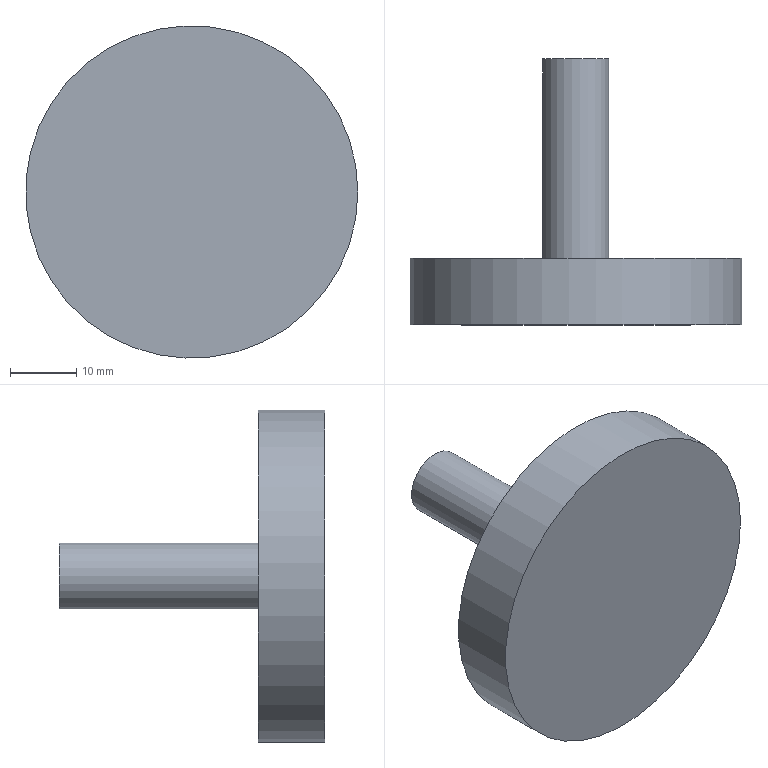Component | NX | BASE_PLATE | 1 solid | 5 faces | box 50 x 40 x 50 mm | volume 21991 mm3 | plane 3 | cylinder 2 | commonest cylinder face diameters 50 x1 10 x1
STEP:
#1=CARTESIAN_POINT('',(0.,0.,0.));
#2=DIRECTION('',(0.,0.,1.));
#3=DIRECTION('',(1.,0.,0.));
#4=AXIS2_PLACEMENT_3D('',#1,#2,#3);
#5=CARTESIAN_POINT('',(25.,-10.,-0.));
#6=VERTEX_POINT('',#5);
#7=CARTESIAN_POINT('',(0.,-10.,0.));
#8=DIRECTION('',(0.,-1.,0.));
#9=DIRECTION('',(1.,0.,-0.));
#10=AXIS2_PLACEMENT_3D('',#7,#8,#9);
#11=CIRCLE('',#10,25.);
#12=CARTESIAN_POINT('',(0.,-10.,0.));
#13=DIRECTION('',(0.,1.,0.));
#14=DIRECTION('',(0.,0.,1.));
#15=AXIS2_PLACEMENT_3D('',#12,#13,#14);
#16=CYLINDRICAL_SURFACE('',#15,25.);
#17=CARTESIAN_POINT('',(7.854,0.));
#18=DIRECTION('',(-1.,0.));
#19=VECTOR('',#18,1.);
#20=LINE('',#17,#19);
#21=(GEOMETRIC_REPRESENTATION_CONTEXT(2)PARAMETRIC_REPRESENTATION_CONTEXT()REPRESENTATION_CONTEXT('',''));
#22=DEFINITIONAL_REPRESENTATION('',(#20),#21);
#23=PCURVE('',#16,#22);
#24=CARTESIAN_POINT('',(0.,-10.,0.));
#25=DIRECTION('',(0.,-1.,0.));
#26=DIRECTION('',(0.,0.,-1.));
#27=AXIS2_PLACEMENT_3D('',#24,#25,#26);
#28=PLANE('',#27);
#29=CARTESIAN_POINT('',(0.,0.));
#30=DIRECTION('',(0.,1.));
#31=AXIS2_PLACEMENT_2D('',#29,#30);
#32=CIRCLE('',#31,25.);
#33=(GEOMETRIC_REPRESENTATION_CONTEXT(2)PARAMETRIC_REPRESENTATION_CONTEXT()REPRESENTATION_CONTEXT('',''));
#34=DEFINITIONAL_REPRESENTATION('',(#32),#33);
#35=PCURVE('',#28,#34);
#36=SURFACE_CURVE('',#11,(#23,#35),.PCURVE_S1.);
#37=EDGE_CURVE('',#6,#6,#36,.T.);
#38=ORIENTED_EDGE('',*,*,#37,.F.);
#39=CARTESIAN_POINT('',(25.,0.,-0.));
#40=VERTEX_POINT('',#39);
#41=CARTESIAN_POINT('',(25.,-10.,0.));
#42=CARTESIAN_POINT('',(25.,0.,0.));
#43=B_SPLINE_CURVE_WITH_KNOTS('',1,(#41,#42),.UNSPECIFIED.,.F.,.F.,(2,2),(0.,10.),.PIECEWISE_BEZIER_KNOTS.);
#44=CARTESIAN_POINT('',(7.854,0.));
#45=DIRECTION('',(0.,1.));
#46=VECTOR('',#45,1.);
#47=LINE('',#44,#46);
#48=(GEOMETRIC_REPRESENTATION_CONTEXT(2)PARAMETRIC_REPRESENTATION_CONTEXT()REPRESENTATION_CONTEXT('',''));
#49=DEFINITIONAL_REPRESENTATION('',(#47),#48);
#50=PCURVE('',#16,#49);
#51=CARTESIAN_POINT('',(1.571,0.));
#52=DIRECTION('',(0.,1.));
#53=VECTOR('',#52,1.);
#54=LINE('',#51,#53);
#55=(GEOMETRIC_REPRESENTATION_CONTEXT(2)PARAMETRIC_REPRESENTATION_CONTEXT()REPRESENTATION_CONTEXT('',''));
#56=DEFINITIONAL_REPRESENTATION('',(#54),#55);
#57=PCURVE('',#16,#56);
#58=SEAM_CURVE('',#43,(#50,#57),.PCURVE_S1.);
#59=EDGE_CURVE('',#6,#40,#58,.T.);
#60=ORIENTED_EDGE('',*,*,#59,.T.);
#61=CARTESIAN_POINT('',(0.,0.,0.));
#62=DIRECTION('',(0.,-1.,0.));
#63=DIRECTION('',(1.,0.,-0.));
#64=AXIS2_PLACEMENT_3D('',#61,#62,#63);
#65=CIRCLE('',#64,25.);
#66=CARTESIAN_POINT('',(7.854,10.));
#67=DIRECTION('',(-1.,0.));
#68=VECTOR('',#67,1.);
#69=LINE('',#66,#68);
#70=(GEOMETRIC_REPRESENTATION_CONTEXT(2)PARAMETRIC_REPRESENTATION_CONTEXT()REPRESENTATION_CONTEXT('',''));
#71=DEFINITIONAL_REPRESENTATION('',(#69),#70);
#72=PCURVE('',#16,#71);
#73=CARTESIAN_POINT('',(0.,0.,0.));
#74=DIRECTION('',(0.,-1.,0.));
#75=DIRECTION('',(0.,0.,-1.));
#76=AXIS2_PLACEMENT_3D('',#73,#74,#75);
#77=PLANE('',#76);
#78=CARTESIAN_POINT('',(0.,0.));
#79=DIRECTION('',(0.,1.));
#80=AXIS2_PLACEMENT_2D('',#78,#79);
#81=CIRCLE('',#80,25.);
#82=(GEOMETRIC_REPRESENTATION_CONTEXT(2)PARAMETRIC_REPRESENTATION_CONTEXT()REPRESENTATION_CONTEXT('',''));
#83=DEFINITIONAL_REPRESENTATION('',(#81),#82);
#84=PCURVE('',#77,#83);
#85=SURFACE_CURVE('',#65,(#72,#84),.PCURVE_S1.);
#86=EDGE_CURVE('',#40,#40,#85,.T.);
#87=ORIENTED_EDGE('',*,*,#86,.T.);
#88=ORIENTED_EDGE('',*,*,#59,.F.);
#89=EDGE_LOOP('',(#38,#60,#87,#88));
#90=FACE_BOUND('',#89,.T.);
#91=ADVANCED_FACE('',(#90),#16,.T.);
#92=ORIENTED_EDGE('',*,*,#37,.T.);
#93=EDGE_LOOP('',(#92));
#94=FACE_BOUND('',#93,.T.);
#95=ADVANCED_FACE('',(#94),#28,.T.);
#96=CARTESIAN_POINT('',(5.,0.,0.));
#97=VERTEX_POINT('',#96);
#98=CARTESIAN_POINT('',(0.,0.,0.));
#99=DIRECTION('',(0.,1.,0.));
#100=DIRECTION('',(1.,0.,0.));
#101=AXIS2_PLACEMENT_3D('',#98,#99,#100);
#102=CIRCLE('',#101,5.);
#103=CARTESIAN_POINT('',(-0.,5.));
#104=CARTESIAN_POINT('',(8.66,5.));
#105=CARTESIAN_POINT('',(4.33,-2.5));
#106=CARTESIAN_POINT('',(0.,-10.));
#107=CARTESIAN_POINT('',(-4.33,-2.5));
#108=CARTESIAN_POINT('',(-8.66,5.));
#109=CARTESIAN_POINT('',(-0.,5.));
#110=(BOUNDED_CURVE()B_SPLINE_CURVE(2,(#103,#104,#105,#106,#107,#108,#109),.UNSPECIFIED.,.T.,.F.)B_SPLINE_CURVE_WITH_KNOTS((1,2,2,2,2,1),(-2.094,0.,2.094,4.189,6.283,8.378),.UNSPECIFIED.)CURVE()GEOMETRIC_REPRESENTATION_ITEM()RATIONAL_B_SPLINE_CURVE((1.,0.5,1.,0.5,1.,0.5,1.))REPRESENTATION_ITEM(''));
#111=(GEOMETRIC_REPRESENTATION_CONTEXT(2)PARAMETRIC_REPRESENTATION_CONTEXT()REPRESENTATION_CONTEXT('',''));
#112=DEFINITIONAL_REPRESENTATION('',(#110),#111);
#113=PCURVE('',#77,#112);
#114=CARTESIAN_POINT('',(0.,30.,0.));
#115=DIRECTION('',(0.,-1.,0.));
#116=DIRECTION('',(0.,0.,-1.));
#117=AXIS2_PLACEMENT_3D('',#114,#115,#116);
#118=CYLINDRICAL_SURFACE('',#117,5.);
#119=CARTESIAN_POINT('',(7.854,30.));
#120=DIRECTION('',(-1.,0.));
#121=VECTOR('',#120,1.);
#122=LINE('',#119,#121);
#123=(GEOMETRIC_REPRESENTATION_CONTEXT(2)PARAMETRIC_REPRESENTATION_CONTEXT()REPRESENTATION_CONTEXT('',''));
#124=DEFINITIONAL_REPRESENTATION('',(#122),#123);
#125=PCURVE('',#118,#124);
#126=SURFACE_CURVE('',#102,(#113,#125),.PCURVE_S1.);
#127=EDGE_CURVE('',#97,#97,#126,.T.);
#128=ORIENTED_EDGE('',*,*,#127,.F.);
#129=EDGE_LOOP('',(#128));
#130=FACE_BOUND('',#129,.T.);
#131=ORIENTED_EDGE('',*,*,#86,.F.);
#132=EDGE_LOOP('',(#131));
#133=FACE_BOUND('',#132,.T.);
#134=ADVANCED_FACE('',(#130,#133),#77,.F.);
#135=CARTESIAN_POINT('',(5.,30.,0.));
#136=VERTEX_POINT('',#135);
#137=CARTESIAN_POINT('',(0.,30.,0.));
#138=DIRECTION('',(0.,1.,0.));
#139=DIRECTION('',(1.,0.,0.));
#140=AXIS2_PLACEMENT_3D('',#137,#138,#139);
#141=CIRCLE('',#140,5.);
#142=CARTESIAN_POINT('',(7.854,0.));
#143=DIRECTION('',(-1.,0.));
#144=VECTOR('',#143,1.);
#145=LINE('',#142,#144);
#146=(GEOMETRIC_REPRESENTATION_CONTEXT(2)PARAMETRIC_REPRESENTATION_CONTEXT()REPRESENTATION_CONTEXT('',''));
#147=DEFINITIONAL_REPRESENTATION('',(#145),#146);
#148=PCURVE('',#118,#147);
#149=CARTESIAN_POINT('',(0.,30.,0.));
#150=DIRECTION('',(0.,1.,0.));
#151=DIRECTION('',(0.,0.,1.));
#152=AXIS2_PLACEMENT_3D('',#149,#150,#151);
#153=PLANE('',#152);
#154=CARTESIAN_POINT('',(0.,0.));
#155=DIRECTION('',(0.,1.));
#156=AXIS2_PLACEMENT_2D('',#154,#155);
#157=CIRCLE('',#156,5.);
#158=(GEOMETRIC_REPRESENTATION_CONTEXT(2)PARAMETRIC_REPRESENTATION_CONTEXT()REPRESENTATION_CONTEXT('',''));
#159=DEFINITIONAL_REPRESENTATION('',(#157),#158);
#160=PCURVE('',#153,#159);
#161=SURFACE_CURVE('',#141,(#148,#160),.PCURVE_S1.);
#162=EDGE_CURVE('',#136,#136,#161,.T.);
#163=ORIENTED_EDGE('',*,*,#162,.F.);
#164=CARTESIAN_POINT('',(5.,30.,-0.));
#165=CARTESIAN_POINT('',(5.,0.,-0.));
#166=B_SPLINE_CURVE_WITH_KNOTS('',1,(#164,#165),.UNSPECIFIED.,.F.,.F.,(2,2),(0.,30.),.PIECEWISE_BEZIER_KNOTS.);
#167=CARTESIAN_POINT('',(7.854,0.));
#168=DIRECTION('',(0.,1.));
#169=VECTOR('',#168,1.);
#170=LINE('',#167,#169);
#171=(GEOMETRIC_REPRESENTATION_CONTEXT(2)PARAMETRIC_REPRESENTATION_CONTEXT()REPRESENTATION_CONTEXT('',''));
#172=DEFINITIONAL_REPRESENTATION('',(#170),#171);
#173=PCURVE('',#118,#172);
#174=CARTESIAN_POINT('',(1.571,0.));
#175=DIRECTION('',(0.,1.));
#176=VECTOR('',#175,1.);
#177=LINE('',#174,#176);
#178=(GEOMETRIC_REPRESENTATION_CONTEXT(2)PARAMETRIC_REPRESENTATION_CONTEXT()REPRESENTATION_CONTEXT('',''));
#179=DEFINITIONAL_REPRESENTATION('',(#177),#178);
#180=PCURVE('',#118,#179);
#181=SEAM_CURVE('',#166,(#173,#180),.PCURVE_S1.);
#182=EDGE_CURVE('',#136,#97,#181,.T.);
#183=ORIENTED_EDGE('',*,*,#182,.T.);
#184=ORIENTED_EDGE('',*,*,#127,.T.);
#185=ORIENTED_EDGE('',*,*,#182,.F.);
#186=EDGE_LOOP('',(#163,#183,#184,#185));
#187=FACE_BOUND('',#186,.T.);
#188=ADVANCED_FACE('',(#187),#118,.T.);
#189=ORIENTED_EDGE('',*,*,#162,.T.);
#190=EDGE_LOOP('',(#189));
#191=FACE_BOUND('',#190,.T.);
#192=ADVANCED_FACE('',(#191),#153,.T.);
#193=CLOSED_SHELL('',(#91,#95,#134,#188,#192));
#194=MANIFOLD_SOLID_BREP('',#193);
#195=(LENGTH_UNIT()NAMED_UNIT(*)SI_UNIT(.MILLI.,.METRE.));
#196=UNCERTAINTY_MEASURE_WITH_UNIT(LENGTH_MEASURE(0.00001),#195,'','');
#197=(NAMED_UNIT(*)PLANE_ANGLE_UNIT()SI_UNIT($,.RADIAN.));
#198=(NAMED_UNIT(*)SI_UNIT($,.STERADIAN.)SOLID_ANGLE_UNIT());
#199=(GEOMETRIC_REPRESENTATION_CONTEXT(3)GLOBAL_UNCERTAINTY_ASSIGNED_CONTEXT((#196))GLOBAL_UNIT_ASSIGNED_CONTEXT((#195,#197,#198))REPRESENTATION_CONTEXT('',''));
#200=ADVANCED_BREP_SHAPE_REPRESENTATION('',(#4,#194),#199);